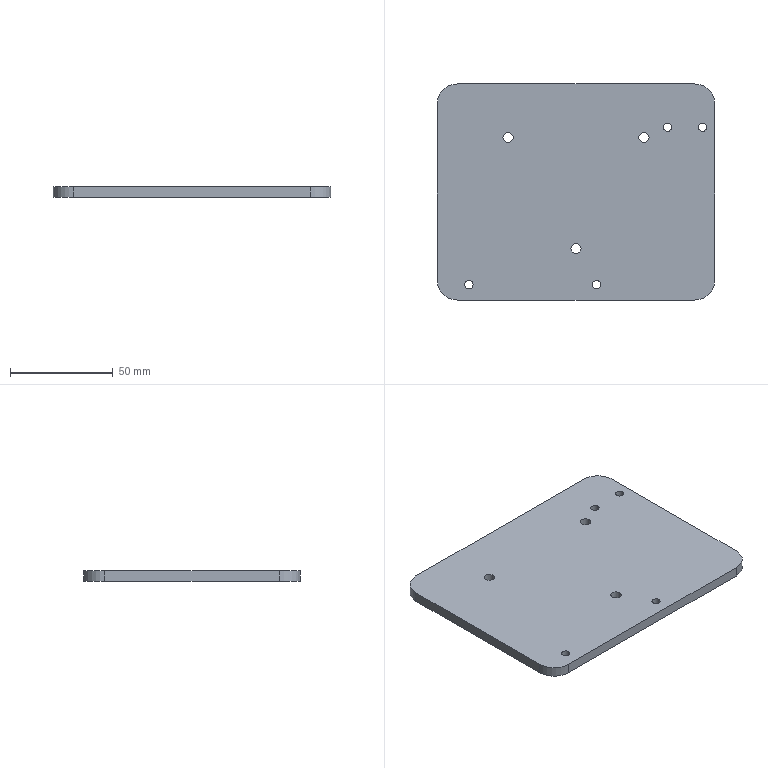Component | NX | BOTTOM_PLATE | 1 solid | 17 faces | volume 69900 mm3 | cylinder 11 | plane 6 | commonest cylinder face diameters 20 x4 4 x4 5 x3